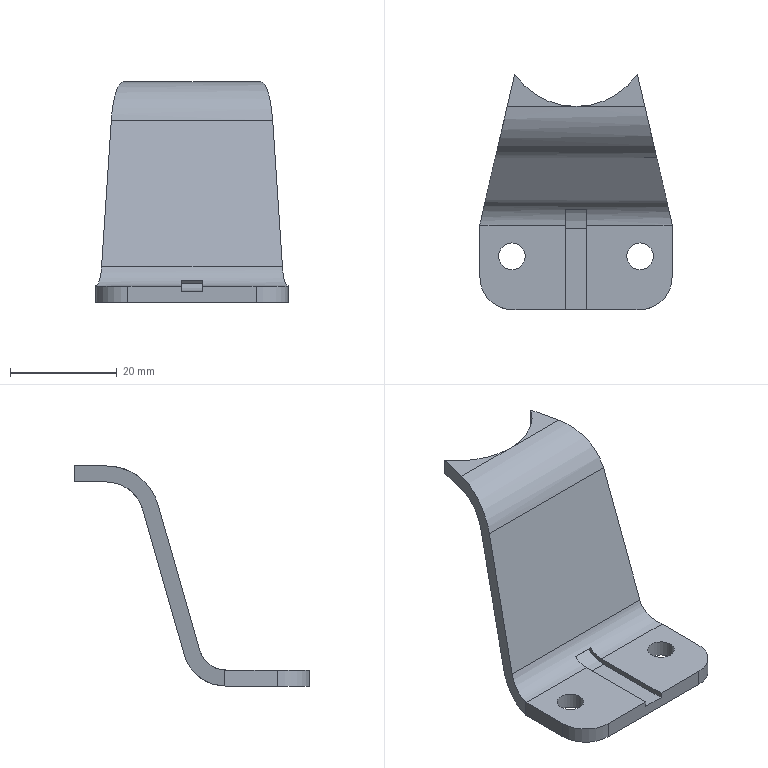Component | NX | 02D__27_3 | 1 solid | 28 faces | volume 6081 mm3 | plane 18 | cylinder 10 | commonest cylinder face diameters 12 x3 5 x2 10 x1 14 x1 16 x1 20 x1 28 x1